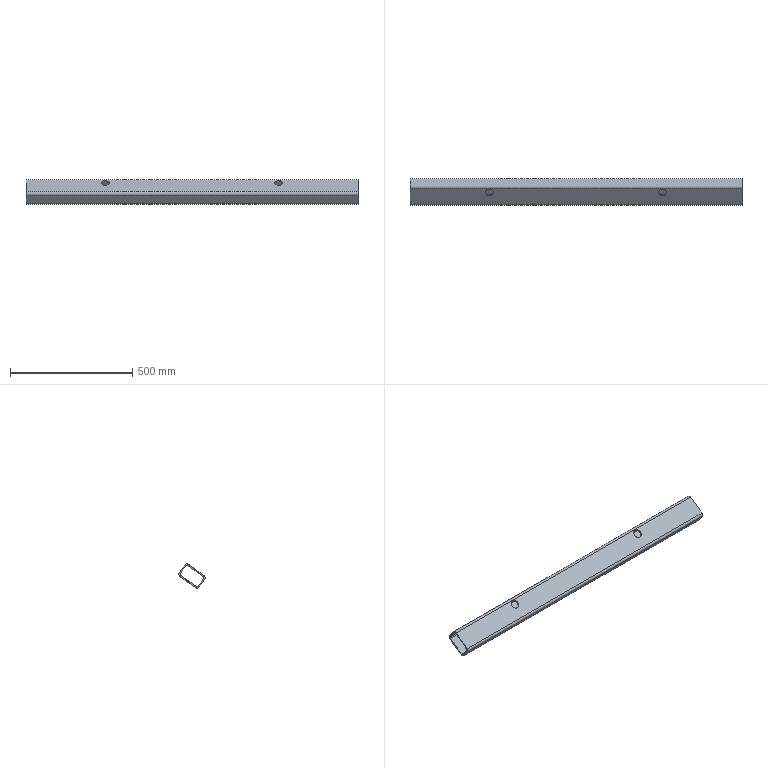Component | SolidWorks | Poprecna spona 1360mm-48 | 1 solid | 26 faces | box 1360 x 108.18 x 99.53 mm | volume 1934284 mm3 | cylinder 16 | plane 10 | commonest cylinder face diameters 34 x8 20 x4 10 x4 | material Plain Carbon Steel
build123d program:
from build123d import *

# Parameters (mm, degrees)
BOSS_EXTRUDE1_DEPTH      = 680
BOSS_EXTRUDE1_DEPTH_BACK = 680
SKETCH2_R                = 17
CUT_EXTRUDE1_DEPTH       = 685.471


with BuildPart() as part:
    # Sketch1 → Boss-Extrude1 (new, two sides: drawn at the far end of the back side and taken through both)
    with BuildSketch(Plane(origin=(0, 0, 0), x_dir=(0, 0, -1), z_dir=(1, 0, 0)).offset(-BOSS_EXTRUDE1_DEPTH_BACK)):
        with BuildLine():
            Line((-20, 50), (20, 50))
            ThreePointArc((20, 50), (27.071, 47.071), (30, 40))
            Line((30, 40), (30, -40))
            ThreePointArc((30, -40), (27.071, -47.071), (20, -50))
            Line((20, -50), (-20, -50))
            ThreePointArc((-20, -50), (-27.071, -47.071), (-30, -40))
            Line((-30, -40), (-30, 40))
            ThreePointArc((-30, 40), (-27.071, 47.071), (-20, 50))
        make_face()
        with BuildLine():
            Line((-25, 40), (-25, -40))
            ThreePointArc((-25, -40), (-23.536, -43.536), (-20, -45))
            Line((-20, -45), (20, -45))
            ThreePointArc((20, -45), (23.536, -43.536), (25, -40))
            Line((25, -40), (25, 40))
            ThreePointArc((25, 40), (23.536, 43.536), (20, 45))
            Line((20, 45), (-20, 45))
            ThreePointArc((-20, 45), (-23.536, 43.536), (-25, 40))
        make_face(mode=Mode.SUBTRACT)
    extrude(amount=BOSS_EXTRUDE1_DEPTH + BOSS_EXTRUDE1_DEPTH_BACK)

    # Sketch2 → Cut-Extrude1 (cut, through all)
    with BuildSketch(Plane.XY.offset(30)):
        with Locations((-355, 20)):
            Circle(SKETCH2_R)
    cut_extrude1 = extrude(amount=-CUT_EXTRUDE1_DEPTH, mode=Mode.SUBTRACT)

    # Mirror1: Cut-Extrude1 across plane
    add(cut_extrude1.mirror(Plane(origin=(0, 0, 0), x_dir=(0, 0, 1), z_dir=(1, 0, 0))), mode=Mode.SUBTRACT)


solid = part.part

# Placed as in the assembly
solid = solid.moved(Location((-633.6, 700.788, 236.028), (36.21, 0, 0)))
STEP:
#1=COLOUR_RGB('',0.7922,0.8196,0.9333);
#2=FILL_AREA_STYLE_COLOUR('',#1);
#3=FILL_AREA_STYLE('',(#2));
#4=SURFACE_STYLE_FILL_AREA(#3);
#5=SURFACE_SIDE_STYLE('',(#4));
#6=SURFACE_STYLE_USAGE(.BOTH.,#5);
#7=PRESENTATION_STYLE_ASSIGNMENT((#6));
#8=CARTESIAN_POINT('',(-10.299,28.923,8.805));
#9=VERTEX_POINT('',#8);
#10=CARTESIAN_POINT('',(-11.638,28.923,8.805));
#11=VERTEX_POINT('',#10);
#12=CARTESIAN_POINT('',(-10.969,28.923,8.805));
#13=DIRECTION('',(-0.,0.5907,-0.8069));
#14=DIRECTION('',(-1.,0.,0.));
#15=AXIS2_PLACEMENT_3D('',#12,#13,#14);
#16=CIRCLE('',#15,0.6693);
#17=EDGE_CURVE('',#9,#11,#16,.T.);
#18=ORIENTED_EDGE('',*,*,#17,.T.);
#19=CARTESIAN_POINT('',(-11.638,28.807,8.963));
#20=VERTEX_POINT('',#19);
#21=CARTESIAN_POINT('',(-11.638,28.923,8.805));
#22=DIRECTION('',(0.,-0.5907,0.8069));
#23=VECTOR('',#22,39.37);
#24=LINE('',#21,#23);
#25=EDGE_CURVE('',#11,#20,#24,.T.);
#26=ORIENTED_EDGE('',*,*,#25,.T.);
#27=CARTESIAN_POINT('',(-10.299,28.807,8.963));
#28=VERTEX_POINT('',#27);
#29=CARTESIAN_POINT('',(-10.969,28.807,8.963));
#30=DIRECTION('',(0.,-0.5907,0.8069));
#31=DIRECTION('',(0.,0.8069,0.5907));
#32=AXIS2_PLACEMENT_3D('',#29,#30,#31);
#33=CIRCLE('',#32,0.6693);
#34=EDGE_CURVE('',#20,#28,#33,.T.);
#35=ORIENTED_EDGE('',*,*,#34,.T.);
#36=CARTESIAN_POINT('',(-10.299,28.923,8.805));
#37=DIRECTION('',(0.,-0.5907,0.8069));
#38=VECTOR('',#37,39.37);
#39=LINE('',#36,#38);
#40=EDGE_CURVE('',#9,#28,#39,.T.);
#41=ORIENTED_EDGE('',*,*,#40,.F.);
#42=EDGE_LOOP('',(#18,#26,#35,#41));
#43=FACE_OUTER_BOUND('',#42,.T.);
#44=CARTESIAN_POINT('',(-10.969,28.923,8.805));
#45=DIRECTION('',(0.,-0.5907,0.8069));
#46=DIRECTION('',(1.,0.,0.));
#47=AXIS2_PLACEMENT_3D('',#44,#45,#46);
#48=CYLINDRICAL_SURFACE('',#47,0.6693);
#49=ADVANCED_FACE('',(#43),#48,.F.);
#50=CARTESIAN_POINT('',(-10.299,27.644,10.552));
#51=VERTEX_POINT('',#50);
#52=CARTESIAN_POINT('',(-11.638,27.644,10.552));
#53=VERTEX_POINT('',#52);
#54=CARTESIAN_POINT('',(-10.969,27.644,10.552));
#55=DIRECTION('',(-0.,0.5907,-0.8069));
#56=DIRECTION('',(1.,0.,0.));
#57=AXIS2_PLACEMENT_3D('',#54,#55,#56);
#58=CIRCLE('',#57,0.6693);
#59=EDGE_CURVE('',#51,#53,#58,.T.);
#60=ORIENTED_EDGE('',*,*,#59,.T.);
#61=CARTESIAN_POINT('',(-11.638,27.528,10.711));
#62=VERTEX_POINT('',#61);
#63=CARTESIAN_POINT('',(-11.638,28.923,8.805));
#64=DIRECTION('',(0.,-0.5907,0.8069));
#65=VECTOR('',#64,39.37);
#66=LINE('',#63,#65);
#67=EDGE_CURVE('',#53,#62,#66,.T.);
#68=ORIENTED_EDGE('',*,*,#67,.T.);
#69=CARTESIAN_POINT('',(-10.299,27.528,10.711));
#70=VERTEX_POINT('',#69);
#71=CARTESIAN_POINT('',(-10.969,27.528,10.711));
#72=DIRECTION('',(-0.,0.5907,-0.8069));
#73=DIRECTION('',(-1.,0.,0.));
#74=AXIS2_PLACEMENT_3D('',#71,#72,#73);
#75=CIRCLE('',#74,0.6693);
#76=EDGE_CURVE('',#70,#62,#75,.T.);
#77=ORIENTED_EDGE('',*,*,#76,.F.);
#78=CARTESIAN_POINT('',(-10.299,28.923,8.805));
#79=DIRECTION('',(0.,-0.5907,0.8069));
#80=VECTOR('',#79,39.37);
#81=LINE('',#78,#80);
#82=EDGE_CURVE('',#51,#70,#81,.T.);
#83=ORIENTED_EDGE('',*,*,#82,.F.);
#84=EDGE_LOOP('',(#60,#68,#77,#83));
#85=FACE_OUTER_BOUND('',#84,.T.);
#86=CARTESIAN_POINT('',(-10.969,28.923,8.805));
#87=DIRECTION('',(0.,-0.5907,0.8069));
#88=DIRECTION('',(1.,0.,0.));
#89=AXIS2_PLACEMENT_3D('',#86,#87,#88);
#90=CYLINDRICAL_SURFACE('',#89,0.6693);
#91=ADVANCED_FACE('',(#85),#90,.F.);
#92=CARTESIAN_POINT('',(-39.591,28.923,8.805));
#93=VERTEX_POINT('',#92);
#94=CARTESIAN_POINT('',(-38.252,28.923,8.805));
#95=VERTEX_POINT('',#94);
#96=CARTESIAN_POINT('',(-38.921,28.923,8.805));
#97=DIRECTION('',(0.,-0.5907,0.8069));
#98=DIRECTION('',(1.,0.,0.));
#99=AXIS2_PLACEMENT_3D('',#96,#97,#98);
#100=CIRCLE('',#99,0.6693);
#101=EDGE_CURVE('',#93,#95,#100,.T.);
#102=ORIENTED_EDGE('',*,*,#101,.F.);
#103=CARTESIAN_POINT('',(-39.591,28.807,8.963));
#104=VERTEX_POINT('',#103);
#105=CARTESIAN_POINT('',(-39.591,28.923,8.805));
#106=DIRECTION('',(0.,-0.5907,0.8069));
#107=VECTOR('',#106,39.37);
#108=LINE('',#105,#107);
#109=EDGE_CURVE('',#93,#104,#108,.T.);
#110=ORIENTED_EDGE('',*,*,#109,.T.);
#111=CARTESIAN_POINT('',(-38.252,28.807,8.963));
#112=VERTEX_POINT('',#111);
#113=CARTESIAN_POINT('',(-38.921,28.807,8.963));
#114=DIRECTION('',(-0.,0.5907,-0.8069));
#115=DIRECTION('',(0.,0.8069,0.5907));
#116=AXIS2_PLACEMENT_3D('',#113,#114,#115);
#117=CIRCLE('',#116,0.6693);
#118=EDGE_CURVE('',#112,#104,#117,.T.);
#119=ORIENTED_EDGE('',*,*,#118,.F.);
#120=CARTESIAN_POINT('',(-38.252,28.923,8.805));
#121=DIRECTION('',(0.,-0.5907,0.8069));
#122=VECTOR('',#121,39.37);
#123=LINE('',#120,#122);
#124=EDGE_CURVE('',#95,#112,#123,.T.);
#125=ORIENTED_EDGE('',*,*,#124,.F.);
#126=EDGE_LOOP('',(#102,#110,#119,#125));
#127=FACE_OUTER_BOUND('',#126,.T.);
#128=CARTESIAN_POINT('',(-38.921,28.923,8.805));
#129=DIRECTION('',(0.,-0.5907,0.8069));
#130=DIRECTION('',(1.,0.,0.));
#131=AXIS2_PLACEMENT_3D('',#128,#129,#130);
#132=CYLINDRICAL_SURFACE('',#131,0.6693);
#133=ADVANCED_FACE('',(#127),#132,.F.);
#134=CARTESIAN_POINT('',(-39.591,27.644,10.552));
#135=VERTEX_POINT('',#134);
#136=CARTESIAN_POINT('',(-38.252,27.644,10.552));
#137=VERTEX_POINT('',#136);
#138=CARTESIAN_POINT('',(-38.921,27.644,10.552));
#139=DIRECTION('',(0.,-0.5907,0.8069));
#140=DIRECTION('',(1.,0.,0.));
#141=AXIS2_PLACEMENT_3D('',#138,#139,#140);
#142=CIRCLE('',#141,0.6693);
#143=EDGE_CURVE('',#135,#137,#142,.T.);
#144=ORIENTED_EDGE('',*,*,#143,.F.);
#145=CARTESIAN_POINT('',(-39.591,27.528,10.711));
#146=VERTEX_POINT('',#145);
#147=CARTESIAN_POINT('',(-39.591,28.923,8.805));
#148=DIRECTION('',(0.,-0.5907,0.8069));
#149=VECTOR('',#148,39.37);
#150=LINE('',#147,#149);
#151=EDGE_CURVE('',#135,#146,#150,.T.);
#152=ORIENTED_EDGE('',*,*,#151,.T.);
#153=CARTESIAN_POINT('',(-38.252,27.528,10.711));
#154=VERTEX_POINT('',#153);
#155=CARTESIAN_POINT('',(-38.921,27.528,10.711));
#156=DIRECTION('',(0.,-0.5907,0.8069));
#157=DIRECTION('',(1.,0.,0.));
#158=AXIS2_PLACEMENT_3D('',#155,#156,#157);
#159=CIRCLE('',#158,0.6693);
#160=EDGE_CURVE('',#146,#154,#159,.T.);
#161=ORIENTED_EDGE('',*,*,#160,.T.);
#162=CARTESIAN_POINT('',(-38.252,28.923,8.805));
#163=DIRECTION('',(0.,-0.5907,0.8069));
#164=VECTOR('',#163,39.37);
#165=LINE('',#162,#164);
#166=EDGE_CURVE('',#137,#154,#165,.T.);
#167=ORIENTED_EDGE('',*,*,#166,.F.);
#168=EDGE_LOOP('',(#144,#152,#161,#167));
#169=FACE_OUTER_BOUND('',#168,.T.);
#170=CARTESIAN_POINT('',(-38.921,28.923,8.805));
#171=DIRECTION('',(0.,-0.5907,0.8069));
#172=DIRECTION('',(1.,0.,0.));
#173=AXIS2_PLACEMENT_3D('',#170,#171,#172);
#174=CYLINDRICAL_SURFACE('',#173,0.6693);
#175=ADVANCED_FACE('',(#169),#174,.F.);
#176=CARTESIAN_POINT('',(-51.717,25.537,8.765));
#177=VERTEX_POINT('',#176);
#178=CARTESIAN_POINT('',(1.827,25.537,8.765));
#179=VERTEX_POINT('',#178);
#180=CARTESIAN_POINT('',(-51.717,25.537,8.765));
#181=DIRECTION('',(1.,-0.,-0.));
#182=VECTOR('',#181,39.37);
#183=LINE('',#180,#182);
#184=EDGE_CURVE('',#177,#179,#183,.T.);
#185=ORIENTED_EDGE('',*,*,#184,.T.);
#186=CARTESIAN_POINT('',(1.827,25.622,9.315));
#187=VERTEX_POINT('',#186);
#188=CARTESIAN_POINT('',(1.827,25.854,8.997));
#189=DIRECTION('',(1.,-0.,-0.));
#190=DIRECTION('',(0.,0.5907,-0.8069));
#191=AXIS2_PLACEMENT_3D('',#188,#189,#190);
#192=CIRCLE('',#191,0.3937);
#193=EDGE_CURVE('',#187,#179,#192,.T.);
#194=ORIENTED_EDGE('',*,*,#193,.F.);
#195=CARTESIAN_POINT('',(-51.717,25.622,9.315));
#196=VERTEX_POINT('',#195);
#197=CARTESIAN_POINT('',(-51.717,25.622,9.315));
#198=DIRECTION('',(1.,-0.,-0.));
#199=VECTOR('',#198,39.37);
#200=LINE('',#197,#199);
#201=EDGE_CURVE('',#196,#187,#200,.T.);
#202=ORIENTED_EDGE('',*,*,#201,.F.);
#203=CARTESIAN_POINT('',(-51.717,25.854,8.997));
#204=DIRECTION('',(1.,-0.,-0.));
#205=DIRECTION('',(0.,0.5907,-0.8069));
#206=AXIS2_PLACEMENT_3D('',#203,#204,#205);
#207=CIRCLE('',#206,0.3937);
#208=EDGE_CURVE('',#196,#177,#207,.T.);
#209=ORIENTED_EDGE('',*,*,#208,.T.);
#210=EDGE_LOOP('',(#185,#194,#202,#209));
#211=FACE_OUTER_BOUND('',#210,.T.);
#212=CARTESIAN_POINT('',(-51.717,25.854,8.997));
#213=DIRECTION('',(1.,-0.,-0.));
#214=DIRECTION('',(0.,0.5907,-0.8069));
#215=AXIS2_PLACEMENT_3D('',#212,#213,#214);
#216=CYLINDRICAL_SURFACE('',#215,0.3937);
#217=ADVANCED_FACE('',(#211),#216,.T.);
#218=ORIENTED_EDGE('',*,*,#76,.T.);
#219=CARTESIAN_POINT('',(-10.969,27.528,10.711));
#220=DIRECTION('',(-0.,0.5907,-0.8069));
#221=DIRECTION('',(-1.,0.,0.));
#222=AXIS2_PLACEMENT_3D('',#219,#220,#221);
#223=CIRCLE('',#222,0.6693);
#224=EDGE_CURVE('',#62,#70,#223,.T.);
#225=ORIENTED_EDGE('',*,*,#224,.T.);
#226=EDGE_LOOP('',(#218,#225));
#227=FACE_BOUND('',#226,.T.);
#228=CARTESIAN_POINT('',(-38.921,27.528,10.711));
#229=DIRECTION('',(0.,-0.5907,0.8069));
#230=DIRECTION('',(1.,0.,0.));
#231=AXIS2_PLACEMENT_3D('',#228,#229,#230);
#232=CIRCLE('',#231,0.6693);
#233=EDGE_CURVE('',#154,#146,#232,.T.);
#234=ORIENTED_EDGE('',*,*,#233,.F.);
#235=ORIENTED_EDGE('',*,*,#160,.F.);
#236=EDGE_LOOP('',(#234,#235));
#237=FACE_BOUND('',#236,.T.);
#238=ORIENTED_EDGE('',*,*,#201,.T.);
#239=CARTESIAN_POINT('',(1.827,28.163,11.176));
#240=VERTEX_POINT('',#239);
#241=CARTESIAN_POINT('',(1.827,28.163,11.176));
#242=DIRECTION('',(-0.,-0.8069,-0.5907));
#243=VECTOR('',#242,39.37);
#244=LINE('',#241,#243);
#245=EDGE_CURVE('',#240,#187,#244,.T.);
#246=ORIENTED_EDGE('',*,*,#245,.F.);
#247=CARTESIAN_POINT('',(-51.717,28.163,11.176));
#248=VERTEX_POINT('',#247);
#249=CARTESIAN_POINT('',(-51.717,28.163,11.176));
#250=DIRECTION('',(1.,-0.,-0.));
#251=VECTOR('',#250,39.37);
#252=LINE('',#249,#251);
#253=EDGE_CURVE('',#248,#240,#252,.T.);
#254=ORIENTED_EDGE('',*,*,#253,.F.);
#255=CARTESIAN_POINT('',(-51.717,28.163,11.176));
#256=DIRECTION('',(-0.,-0.8069,-0.5907));
#257=VECTOR('',#256,39.37);
#258=LINE('',#255,#257);
#259=EDGE_CURVE('',#248,#196,#258,.T.);
#260=ORIENTED_EDGE('',*,*,#259,.T.);
#261=EDGE_LOOP('',(#238,#246,#254,#260));
#262=FACE_OUTER_BOUND('',#261,.T.);
#263=CARTESIAN_POINT('',(-51.717,28.163,11.176));
#264=DIRECTION('',(0.,-0.5907,0.8069));
#265=DIRECTION('',(-0.,-0.8069,-0.5907));
#266=AXIS2_PLACEMENT_3D('',#263,#264,#265);
#267=PLANE('',#266);
#268=ADVANCED_FACE('',(#227,#237,#262),#267,.T.);
#269=ORIENTED_EDGE('',*,*,#253,.T.);
#270=CARTESIAN_POINT('',(1.827,28.713,11.091));
#271=VERTEX_POINT('',#270);
#272=CARTESIAN_POINT('',(1.827,28.396,10.858));
#273=DIRECTION('',(1.,-0.,-0.));
#274=DIRECTION('',(0.,0.5907,-0.8069));
#275=AXIS2_PLACEMENT_3D('',#272,#273,#274);
#276=CIRCLE('',#275,0.3937);
#277=EDGE_CURVE('',#271,#240,#276,.T.);
#278=ORIENTED_EDGE('',*,*,#277,.F.);
#279=CARTESIAN_POINT('',(-51.717,28.713,11.091));
#280=VERTEX_POINT('',#279);
#281=CARTESIAN_POINT('',(-51.717,28.713,11.091));
#282=DIRECTION('',(1.,-0.,-0.));
#283=VECTOR('',#282,39.37);
#284=LINE('',#281,#283);
#285=EDGE_CURVE('',#280,#271,#284,.T.);
#286=ORIENTED_EDGE('',*,*,#285,.F.);
#287=CARTESIAN_POINT('',(-51.717,28.396,10.858));
#288=DIRECTION('',(1.,-0.,-0.));
#289=DIRECTION('',(0.,0.5907,-0.8069));
#290=AXIS2_PLACEMENT_3D('',#287,#288,#289);
#291=CIRCLE('',#290,0.3937);
#292=EDGE_CURVE('',#280,#248,#291,.T.);
#293=ORIENTED_EDGE('',*,*,#292,.T.);
#294=EDGE_LOOP('',(#269,#278,#286,#293));
#295=FACE_OUTER_BOUND('',#294,.T.);
#296=CARTESIAN_POINT('',(-51.717,28.396,10.858));
#297=DIRECTION('',(1.,-0.,-0.));
#298=DIRECTION('',(0.,0.5907,-0.8069));
#299=AXIS2_PLACEMENT_3D('',#296,#297,#298);
#300=CYLINDRICAL_SURFACE('',#299,0.3937);
#301=ADVANCED_FACE('',(#295),#300,.T.);
#302=ORIENTED_EDGE('',*,*,#285,.T.);
#303=CARTESIAN_POINT('',(1.827,29.644,9.82));
#304=VERTEX_POINT('',#303);
#305=CARTESIAN_POINT('',(1.827,28.713,11.091));
#306=DIRECTION('',(0.,-0.5907,0.8069));
#307=VECTOR('',#306,39.37);
#308=LINE('',#305,#307);
#309=EDGE_CURVE('',#304,#271,#308,.T.);
#310=ORIENTED_EDGE('',*,*,#309,.F.);
#311=CARTESIAN_POINT('',(-51.717,29.644,9.82));
#312=VERTEX_POINT('',#311);
#313=CARTESIAN_POINT('',(-51.717,29.644,9.82));
#314=DIRECTION('',(1.,-0.,-0.));
#315=VECTOR('',#314,39.37);
#316=LINE('',#313,#315);
#317=EDGE_CURVE('',#312,#304,#316,.T.);
#318=ORIENTED_EDGE('',*,*,#317,.F.);
#319=CARTESIAN_POINT('',(-51.717,28.713,11.091));
#320=DIRECTION('',(0.,-0.5907,0.8069));
#321=VECTOR('',#320,39.37);
#322=LINE('',#319,#321);
#323=EDGE_CURVE('',#312,#280,#322,.T.);
#324=ORIENTED_EDGE('',*,*,#323,.T.);
#325=EDGE_LOOP('',(#302,#310,#318,#324));
#326=FACE_OUTER_BOUND('',#325,.T.);
#327=CARTESIAN_POINT('',(-51.717,28.713,11.091));
#328=DIRECTION('',(0.,0.8069,0.5907));
#329=DIRECTION('',(0.,-0.5907,0.8069));
#330=AXIS2_PLACEMENT_3D('',#327,#328,#329);
#331=PLANE('',#330);
#332=ADVANCED_FACE('',(#326),#331,.T.);
#333=ORIENTED_EDGE('',*,*,#317,.T.);
#334=CARTESIAN_POINT('',(1.827,29.558,9.27));
#335=VERTEX_POINT('',#334);
#336=CARTESIAN_POINT('',(1.827,29.326,9.587));
#337=DIRECTION('',(1.,-0.,-0.));
#338=DIRECTION('',(0.,-0.5907,0.8069));
#339=AXIS2_PLACEMENT_3D('',#336,#337,#338);
#340=CIRCLE('',#339,0.3937);
#341=EDGE_CURVE('',#335,#304,#340,.T.);
#342=ORIENTED_EDGE('',*,*,#341,.F.);
#343=CARTESIAN_POINT('',(-51.717,29.558,9.27));
#344=VERTEX_POINT('',#343);
#345=CARTESIAN_POINT('',(-51.717,29.558,9.27));
#346=DIRECTION('',(1.,-0.,-0.));
#347=VECTOR('',#346,39.37);
#348=LINE('',#345,#347);
#349=EDGE_CURVE('',#344,#335,#348,.T.);
#350=ORIENTED_EDGE('',*,*,#349,.F.);
#351=CARTESIAN_POINT('',(-51.717,29.326,9.587));
#352=DIRECTION('',(1.,-0.,-0.));
#353=DIRECTION('',(0.,-0.5907,0.8069));
#354=AXIS2_PLACEMENT_3D('',#351,#352,#353);
#355=CIRCLE('',#354,0.3937);
#356=EDGE_CURVE('',#344,#312,#355,.T.);
#357=ORIENTED_EDGE('',*,*,#356,.T.);
#358=EDGE_LOOP('',(#333,#342,#350,#357));
#359=FACE_OUTER_BOUND('',#358,.T.);
#360=CARTESIAN_POINT('',(-51.717,29.326,9.587));
#361=DIRECTION('',(1.,-0.,-0.));
#362=DIRECTION('',(0.,0.5907,-0.8069));
#363=AXIS2_PLACEMENT_3D('',#360,#361,#362);
#364=CYLINDRICAL_SURFACE('',#363,0.3937);
#365=ADVANCED_FACE('',(#359),#364,.T.);
#366=ORIENTED_EDGE('',*,*,#17,.F.);
#367=CARTESIAN_POINT('',(-10.969,28.923,8.805));
#368=DIRECTION('',(-0.,0.5907,-0.8069));
#369=DIRECTION('',(-1.,0.,0.));
#370=AXIS2_PLACEMENT_3D('',#367,#368,#369);
#371=CIRCLE('',#370,0.6693);
#372=EDGE_CURVE('',#11,#9,#371,.T.);
#373=ORIENTED_EDGE('',*,*,#372,.F.);
#374=EDGE_LOOP('',(#366,#373));
#375=FACE_BOUND('',#374,.T.);
#376=CARTESIAN_POINT('',(-38.921,28.923,8.805));
#377=DIRECTION('',(0.,-0.5907,0.8069));
#378=DIRECTION('',(1.,0.,0.));
#379=AXIS2_PLACEMENT_3D('',#376,#377,#378);
#380=CIRCLE('',#379,0.6693);
#381=EDGE_CURVE('',#95,#93,#380,.T.);
#382=ORIENTED_EDGE('',*,*,#381,.T.);
#383=ORIENTED_EDGE('',*,*,#101,.T.);
#384=EDGE_LOOP('',(#382,#383));
#385=FACE_BOUND('',#384,.T.);
#386=ORIENTED_EDGE('',*,*,#349,.T.);
#387=CARTESIAN_POINT('',(1.827,27.017,7.409));
#388=VERTEX_POINT('',#387);
#389=CARTESIAN_POINT('',(1.827,29.558,9.27));
#390=DIRECTION('',(0.,0.8069,0.5907));
#391=VECTOR('',#390,39.37);
#392=LINE('',#389,#391);
#393=EDGE_CURVE('',#388,#335,#392,.T.);
#394=ORIENTED_EDGE('',*,*,#393,.F.);
#395=CARTESIAN_POINT('',(-51.717,27.017,7.409));
#396=VERTEX_POINT('',#395);
#397=CARTESIAN_POINT('',(-51.717,27.017,7.409));
#398=DIRECTION('',(1.,-0.,-0.));
#399=VECTOR('',#398,39.37);
#400=LINE('',#397,#399);
#401=EDGE_CURVE('',#396,#388,#400,.T.);
#402=ORIENTED_EDGE('',*,*,#401,.F.);
#403=CARTESIAN_POINT('',(-51.717,29.558,9.27));
#404=DIRECTION('',(0.,0.8069,0.5907));
#405=VECTOR('',#404,39.37);
#406=LINE('',#403,#405);
#407=EDGE_CURVE('',#396,#344,#406,.T.);
#408=ORIENTED_EDGE('',*,*,#407,.T.);
#409=EDGE_LOOP('',(#386,#394,#402,#408));
#410=FACE_OUTER_BOUND('',#409,.T.);
#411=CARTESIAN_POINT('',(-51.717,29.558,9.27));
#412=DIRECTION('',(-0.,0.5907,-0.8069));
#413=DIRECTION('',(0.,0.8069,0.5907));
#414=AXIS2_PLACEMENT_3D('',#411,#412,#413);
#415=PLANE('',#414);
#416=ADVANCED_FACE('',(#375,#385,#410),#415,.T.);
#417=ORIENTED_EDGE('',*,*,#401,.T.);
#418=CARTESIAN_POINT('',(1.827,26.467,7.494));
#419=VERTEX_POINT('',#418);
#420=CARTESIAN_POINT('',(1.827,26.785,7.727));
#421=DIRECTION('',(1.,-0.,-0.));
#422=DIRECTION('',(0.,0.5907,-0.8069));
#423=AXIS2_PLACEMENT_3D('',#420,#421,#422);
#424=CIRCLE('',#423,0.3937);
#425=EDGE_CURVE('',#419,#388,#424,.T.);
#426=ORIENTED_EDGE('',*,*,#425,.F.);
#427=CARTESIAN_POINT('',(-51.717,26.467,7.494));
#428=VERTEX_POINT('',#427);
#429=CARTESIAN_POINT('',(-51.717,26.467,7.494));
#430=DIRECTION('',(1.,-0.,-0.));
#431=VECTOR('',#430,39.37);
#432=LINE('',#429,#431);
#433=EDGE_CURVE('',#428,#419,#432,.T.);
#434=ORIENTED_EDGE('',*,*,#433,.F.);
#435=CARTESIAN_POINT('',(-51.717,26.785,7.727));
#436=DIRECTION('',(1.,-0.,-0.));
#437=DIRECTION('',(0.,0.5907,-0.8069));
#438=AXIS2_PLACEMENT_3D('',#435,#436,#437);
#439=CIRCLE('',#438,0.3937);
#440=EDGE_CURVE('',#428,#396,#439,.T.);
#441=ORIENTED_EDGE('',*,*,#440,.T.);
#442=EDGE_LOOP('',(#417,#426,#434,#441));
#443=FACE_OUTER_BOUND('',#442,.T.);
#444=CARTESIAN_POINT('',(-51.717,26.785,7.727));
#445=DIRECTION('',(1.,-0.,-0.));
#446=DIRECTION('',(0.,0.5907,-0.8069));
#447=AXIS2_PLACEMENT_3D('',#444,#445,#446);
#448=CYLINDRICAL_SURFACE('',#447,0.3937);
#449=ADVANCED_FACE('',(#443),#448,.T.);
#450=ORIENTED_EDGE('',*,*,#433,.T.);
#451=CARTESIAN_POINT('',(1.827,25.537,8.765));
#452=DIRECTION('',(-0.,0.5907,-0.8069));
#453=VECTOR('',#452,39.37);
#454=LINE('',#451,#453);
#455=EDGE_CURVE('',#179,#419,#454,.T.);
#456=ORIENTED_EDGE('',*,*,#455,.F.);
#457=ORIENTED_EDGE('',*,*,#184,.F.);
#458=CARTESIAN_POINT('',(-51.717,25.537,8.765));
#459=DIRECTION('',(-0.,0.5907,-0.8069));
#460=VECTOR('',#459,39.37);
#461=LINE('',#458,#460);
#462=EDGE_CURVE('',#177,#428,#461,.T.);
#463=ORIENTED_EDGE('',*,*,#462,.T.);
#464=EDGE_LOOP('',(#450,#456,#457,#463));
#465=FACE_OUTER_BOUND('',#464,.T.);
#466=CARTESIAN_POINT('',(-51.717,25.537,8.765));
#467=DIRECTION('',(-0.,-0.8069,-0.5907));
#468=DIRECTION('',(-0.,0.5907,-0.8069));
#469=AXIS2_PLACEMENT_3D('',#466,#467,#468);
#470=PLANE('',#469);
#471=ADVANCED_FACE('',(#465),#470,.T.);
#472=CARTESIAN_POINT('',(-51.717,29.485,9.704));
#473=VERTEX_POINT('',#472);
#474=CARTESIAN_POINT('',(-51.717,28.554,10.974));
#475=VERTEX_POINT('',#474);
#476=CARTESIAN_POINT('',(-51.717,28.554,10.974));
#477=DIRECTION('',(0.,-0.5907,0.8069));
#478=VECTOR('',#477,39.37);
#479=LINE('',#476,#478);
#480=EDGE_CURVE('',#473,#475,#479,.T.);
#481=ORIENTED_EDGE('',*,*,#480,.T.);
#482=CARTESIAN_POINT('',(-51.717,28.279,11.017));
#483=VERTEX_POINT('',#482);
#484=CARTESIAN_POINT('',(-51.717,28.396,10.858));
#485=DIRECTION('',(1.,-0.,-0.));
#486=DIRECTION('',(0.,0.5907,-0.8069));
#487=AXIS2_PLACEMENT_3D('',#484,#485,#486);
#488=CIRCLE('',#487,0.1969);
#489=EDGE_CURVE('',#475,#483,#488,.T.);
#490=ORIENTED_EDGE('',*,*,#489,.T.);
#491=CARTESIAN_POINT('',(-51.717,25.738,9.156));
#492=VERTEX_POINT('',#491);
#493=CARTESIAN_POINT('',(-51.717,28.279,11.017));
#494=DIRECTION('',(-0.,-0.8069,-0.5907));
#495=VECTOR('',#494,39.37);
#496=LINE('',#493,#495);
#497=EDGE_CURVE('',#483,#492,#496,.T.);
#498=ORIENTED_EDGE('',*,*,#497,.T.);
#499=CARTESIAN_POINT('',(-51.717,25.695,8.881));
#500=VERTEX_POINT('',#499);
#501=CARTESIAN_POINT('',(-51.717,25.854,8.997));
#502=DIRECTION('',(1.,-0.,-0.));
#503=DIRECTION('',(0.,0.5907,-0.8069));
#504=AXIS2_PLACEMENT_3D('',#501,#502,#503);
#505=CIRCLE('',#504,0.1969);
#506=EDGE_CURVE('',#492,#500,#505,.T.);
#507=ORIENTED_EDGE('',*,*,#506,.T.);
#508=CARTESIAN_POINT('',(-51.717,26.626,7.611));
#509=VERTEX_POINT('',#508);
#510=CARTESIAN_POINT('',(-51.717,25.695,8.881));
#511=DIRECTION('',(-0.,0.5907,-0.8069));
#512=VECTOR('',#511,39.37);
#513=LINE('',#510,#512);
#514=EDGE_CURVE('',#500,#509,#513,.T.);
#515=ORIENTED_EDGE('',*,*,#514,.T.);
#516=CARTESIAN_POINT('',(-51.717,26.901,7.568));
#517=VERTEX_POINT('',#516);
#518=CARTESIAN_POINT('',(-51.717,26.785,7.727));
#519=DIRECTION('',(1.,-0.,-0.));
#520=DIRECTION('',(0.,0.5907,-0.8069));
#521=AXIS2_PLACEMENT_3D('',#518,#519,#520);
#522=CIRCLE('',#521,0.1969);
#523=EDGE_CURVE('',#509,#517,#522,.T.);
#524=ORIENTED_EDGE('',*,*,#523,.T.);
#525=CARTESIAN_POINT('',(-51.717,29.442,9.429));
#526=VERTEX_POINT('',#525);
#527=CARTESIAN_POINT('',(-51.717,29.442,9.429));
#528=DIRECTION('',(0.,0.8069,0.5907));
#529=VECTOR('',#528,39.37);
#530=LINE('',#527,#529);
#531=EDGE_CURVE('',#517,#526,#530,.T.);
#532=ORIENTED_EDGE('',*,*,#531,.T.);
#533=CARTESIAN_POINT('',(-51.717,29.326,9.587));
#534=DIRECTION('',(1.,-0.,-0.));
#535=DIRECTION('',(0.,-0.5907,0.8069));
#536=AXIS2_PLACEMENT_3D('',#533,#534,#535);
#537=CIRCLE('',#536,0.1969);
#538=EDGE_CURVE('',#526,#473,#537,.T.);
#539=ORIENTED_EDGE('',*,*,#538,.T.);
#540=EDGE_LOOP('',(#481,#490,#498,#507,#515,#524,#532,#539));
#541=FACE_BOUND('',#540,.T.);
#542=ORIENTED_EDGE('',*,*,#208,.F.);
#543=ORIENTED_EDGE('',*,*,#259,.F.);
#544=ORIENTED_EDGE('',*,*,#292,.F.);
#545=ORIENTED_EDGE('',*,*,#323,.F.);
#546=ORIENTED_EDGE('',*,*,#356,.F.);
#547=ORIENTED_EDGE('',*,*,#407,.F.);
#548=ORIENTED_EDGE('',*,*,#440,.F.);
#549=ORIENTED_EDGE('',*,*,#462,.F.);
#550=EDGE_LOOP('',(#542,#543,#544,#545,#546,#547,#548,#549));
#551=FACE_OUTER_BOUND('',#550,.T.);
#552=CARTESIAN_POINT('',(-51.717,25.854,8.997));
#553=DIRECTION('',(1.,-0.,-0.));
#554=DIRECTION('',(-0.,0.5907,-0.8069));
#555=AXIS2_PLACEMENT_3D('',#552,#553,#554);
#556=PLANE('',#555);
#557=ADVANCED_FACE('',(#541,#551),#556,.F.);
#558=CARTESIAN_POINT('',(1.827,28.554,10.974));
#559=VERTEX_POINT('',#558);
#560=CARTESIAN_POINT('',(-51.717,28.554,10.974));
#561=DIRECTION('',(1.,-0.,-0.));
#562=VECTOR('',#561,39.37);
#563=LINE('',#560,#562);
#564=EDGE_CURVE('',#475,#559,#563,.T.);
#565=ORIENTED_EDGE('',*,*,#564,.T.);
#566=CARTESIAN_POINT('',(1.827,28.279,11.017));
#567=VERTEX_POINT('',#566);
#568=CARTESIAN_POINT('',(1.827,28.396,10.858));
#569=DIRECTION('',(1.,-0.,-0.));
#570=DIRECTION('',(0.,0.5907,-0.8069));
#571=AXIS2_PLACEMENT_3D('',#568,#569,#570);
#572=CIRCLE('',#571,0.1969);
#573=EDGE_CURVE('',#559,#567,#572,.T.);
#574=ORIENTED_EDGE('',*,*,#573,.T.);
#575=CARTESIAN_POINT('',(-51.717,28.279,11.017));
#576=DIRECTION('',(1.,-0.,-0.));
#577=VECTOR('',#576,39.37);
#578=LINE('',#575,#577);
#579=EDGE_CURVE('',#483,#567,#578,.T.);
#580=ORIENTED_EDGE('',*,*,#579,.F.);
#581=ORIENTED_EDGE('',*,*,#489,.F.);
#582=EDGE_LOOP('',(#565,#574,#580,#581));
#583=FACE_OUTER_BOUND('',#582,.T.);
#584=CARTESIAN_POINT('',(-51.717,28.396,10.858));
#585=DIRECTION('',(1.,-0.,-0.));
#586=DIRECTION('',(0.,0.5907,-0.8069));
#587=AXIS2_PLACEMENT_3D('',#584,#585,#586);
#588=CYLINDRICAL_SURFACE('',#587,0.1969);
#589=ADVANCED_FACE('',(#583),#588,.F.);
#590=CARTESIAN_POINT('',(1.827,29.485,9.704));
#591=VERTEX_POINT('',#590);
#592=CARTESIAN_POINT('',(-51.717,29.485,9.704));
#593=DIRECTION('',(1.,-0.,-0.));
#594=VECTOR('',#593,39.37);
#595=LINE('',#592,#594);
#596=EDGE_CURVE('',#473,#591,#595,.T.);
#597=ORIENTED_EDGE('',*,*,#596,.T.);
#598=CARTESIAN_POINT('',(1.827,28.554,10.974));
#599=DIRECTION('',(0.,-0.5907,0.8069));
#600=VECTOR('',#599,39.37);
#601=LINE('',#598,#600);
#602=EDGE_CURVE('',#591,#559,#601,.T.);
#603=ORIENTED_EDGE('',*,*,#602,.T.);
#604=ORIENTED_EDGE('',*,*,#564,.F.);
#605=ORIENTED_EDGE('',*,*,#480,.F.);
#606=EDGE_LOOP('',(#597,#603,#604,#605));
#607=FACE_OUTER_BOUND('',#606,.T.);
#608=CARTESIAN_POINT('',(-51.717,28.554,10.974));
#609=DIRECTION('',(0.,0.8069,0.5907));
#610=DIRECTION('',(0.,-0.5907,0.8069));
#611=AXIS2_PLACEMENT_3D('',#608,#609,#610);
#612=PLANE('',#611);
#613=ADVANCED_FACE('',(#607),#612,.F.);
#614=CARTESIAN_POINT('',(1.827,29.442,9.429));
#615=VERTEX_POINT('',#614);
#616=CARTESIAN_POINT('',(-51.717,29.442,9.429));
#617=DIRECTION('',(1.,-0.,-0.));
#618=VECTOR('',#617,39.37);
#619=LINE('',#616,#618);
#620=EDGE_CURVE('',#526,#615,#619,.T.);
#621=ORIENTED_EDGE('',*,*,#620,.T.);
#622=CARTESIAN_POINT('',(1.827,29.326,9.587));
#623=DIRECTION('',(1.,-0.,-0.));
#624=DIRECTION('',(0.,-0.5907,0.8069));
#625=AXIS2_PLACEMENT_3D('',#622,#623,#624);
#626=CIRCLE('',#625,0.1969);
#627=EDGE_CURVE('',#615,#591,#626,.T.);
#628=ORIENTED_EDGE('',*,*,#627,.T.);
#629=ORIENTED_EDGE('',*,*,#596,.F.);
#630=ORIENTED_EDGE('',*,*,#538,.F.);
#631=EDGE_LOOP('',(#621,#628,#629,#630));
#632=FACE_OUTER_BOUND('',#631,.T.);
#633=CARTESIAN_POINT('',(-51.717,29.326,9.587));
#634=DIRECTION('',(1.,-0.,-0.));
#635=DIRECTION('',(0.,0.5907,-0.8069));
#636=AXIS2_PLACEMENT_3D('',#633,#634,#635);
#637=CYLINDRICAL_SURFACE('',#636,0.1969);
#638=ADVANCED_FACE('',(#632),#637,.F.);
#639=CARTESIAN_POINT('',(-10.969,28.807,8.963));
#640=DIRECTION('',(0.,-0.5907,0.8069));
#641=DIRECTION('',(-0.,0.8069,0.5907));
#642=AXIS2_PLACEMENT_3D('',#639,#640,#641);
#643=CIRCLE('',#642,0.6693);
#644=EDGE_CURVE('',#28,#20,#643,.T.);
#645=ORIENTED_EDGE('',*,*,#644,.F.);
#646=ORIENTED_EDGE('',*,*,#34,.F.);
#647=EDGE_LOOP('',(#645,#646));
#648=FACE_BOUND('',#647,.T.);
#649=ORIENTED_EDGE('',*,*,#118,.T.);
#650=CARTESIAN_POINT('',(-38.921,28.807,8.963));
#651=DIRECTION('',(-0.,0.5907,-0.8069));
#652=DIRECTION('',(0.,0.8069,0.5907));
#653=AXIS2_PLACEMENT_3D('',#650,#651,#652);
#654=CIRCLE('',#653,0.6693);
#655=EDGE_CURVE('',#104,#112,#654,.T.);
#656=ORIENTED_EDGE('',*,*,#655,.T.);
#657=EDGE_LOOP('',(#649,#656));
#658=FACE_BOUND('',#657,.T.);
#659=CARTESIAN_POINT('',(1.827,26.901,7.568));
#660=VERTEX_POINT('',#659);
#661=CARTESIAN_POINT('',(-51.717,26.901,7.568));
#662=DIRECTION('',(1.,-0.,-0.));
#663=VECTOR('',#662,39.37);
#664=LINE('',#661,#663);
#665=EDGE_CURVE('',#517,#660,#664,.T.);
#666=ORIENTED_EDGE('',*,*,#665,.T.);
#667=CARTESIAN_POINT('',(1.827,29.442,9.429));
#668=DIRECTION('',(0.,0.8069,0.5907));
#669=VECTOR('',#668,39.37);
#670=LINE('',#667,#669);
#671=EDGE_CURVE('',#660,#615,#670,.T.);
#672=ORIENTED_EDGE('',*,*,#671,.T.);
#673=ORIENTED_EDGE('',*,*,#620,.F.);
#674=ORIENTED_EDGE('',*,*,#531,.F.);
#675=EDGE_LOOP('',(#666,#672,#673,#674));
#676=FACE_OUTER_BOUND('',#675,.T.);
#677=CARTESIAN_POINT('',(-51.717,29.442,9.429));
#678=DIRECTION('',(-0.,0.5907,-0.8069));
#679=DIRECTION('',(0.,0.8069,0.5907));
#680=AXIS2_PLACEMENT_3D('',#677,#678,#679);
#681=PLANE('',#680);
#682=ADVANCED_FACE('',(#648,#658,#676),#681,.F.);
#683=CARTESIAN_POINT('',(1.827,26.626,7.611));
#684=VERTEX_POINT('',#683);
#685=CARTESIAN_POINT('',(-51.717,26.626,7.611));
#686=DIRECTION('',(1.,-0.,-0.));
#687=VECTOR('',#686,39.37);
#688=LINE('',#685,#687);
#689=EDGE_CURVE('',#509,#684,#688,.T.);
#690=ORIENTED_EDGE('',*,*,#689,.T.);
#691=CARTESIAN_POINT('',(1.827,26.785,7.727));
#692=DIRECTION('',(1.,-0.,-0.));
#693=DIRECTION('',(0.,0.5907,-0.8069));
#694=AXIS2_PLACEMENT_3D('',#691,#692,#693);
#695=CIRCLE('',#694,0.1969);
#696=EDGE_CURVE('',#684,#660,#695,.T.);
#697=ORIENTED_EDGE('',*,*,#696,.T.);
#698=ORIENTED_EDGE('',*,*,#665,.F.);
#699=ORIENTED_EDGE('',*,*,#523,.F.);
#700=EDGE_LOOP('',(#690,#697,#698,#699));
#701=FACE_OUTER_BOUND('',#700,.T.);
#702=CARTESIAN_POINT('',(-51.717,26.785,7.727));
#703=DIRECTION('',(1.,-0.,-0.));
#704=DIRECTION('',(0.,0.5907,-0.8069));
#705=AXIS2_PLACEMENT_3D('',#702,#703,#704);
#706=CYLINDRICAL_SURFACE('',#705,0.1969);
#707=ADVANCED_FACE('',(#701),#706,.F.);
#708=CARTESIAN_POINT('',(1.827,25.695,8.881));
#709=VERTEX_POINT('',#708);
#710=CARTESIAN_POINT('',(-51.717,25.695,8.881));
#711=DIRECTION('',(1.,-0.,-0.));
#712=VECTOR('',#711,39.37);
#713=LINE('',#710,#712);
#714=EDGE_CURVE('',#500,#709,#713,.T.);
#715=ORIENTED_EDGE('',*,*,#714,.T.);
#716=CARTESIAN_POINT('',(1.827,25.695,8.881));
#717=DIRECTION('',(-0.,0.5907,-0.8069));
#718=VECTOR('',#717,39.37);
#719=LINE('',#716,#718);
#720=EDGE_CURVE('',#709,#684,#719,.T.);
#721=ORIENTED_EDGE('',*,*,#720,.T.);
#722=ORIENTED_EDGE('',*,*,#689,.F.);
#723=ORIENTED_EDGE('',*,*,#514,.F.);
#724=EDGE_LOOP('',(#715,#721,#722,#723));
#725=FACE_OUTER_BOUND('',#724,.T.);
#726=CARTESIAN_POINT('',(-51.717,25.695,8.881));
#727=DIRECTION('',(-0.,-0.8069,-0.5907));
#728=DIRECTION('',(-0.,0.5907,-0.8069));
#729=AXIS2_PLACEMENT_3D('',#726,#727,#728);
#730=PLANE('',#729);
#731=ADVANCED_FACE('',(#725),#730,.F.);
#732=CARTESIAN_POINT('',(1.827,25.738,9.156));
#733=VERTEX_POINT('',#732);
#734=CARTESIAN_POINT('',(-51.717,25.738,9.156));
#735=DIRECTION('',(1.,-0.,-0.));
#736=VECTOR('',#735,39.37);
#737=LINE('',#734,#736);
#738=EDGE_CURVE('',#492,#733,#737,.T.);
#739=ORIENTED_EDGE('',*,*,#738,.T.);
#740=CARTESIAN_POINT('',(1.827,25.854,8.997));
#741=DIRECTION('',(1.,-0.,-0.));
#742=DIRECTION('',(0.,0.5907,-0.8069));
#743=AXIS2_PLACEMENT_3D('',#740,#741,#742);
#744=CIRCLE('',#743,0.1969);
#745=EDGE_CURVE('',#733,#709,#744,.T.);
#746=ORIENTED_EDGE('',*,*,#745,.T.);
#747=ORIENTED_EDGE('',*,*,#714,.F.);
#748=ORIENTED_EDGE('',*,*,#506,.F.);
#749=EDGE_LOOP('',(#739,#746,#747,#748));
#750=FACE_OUTER_BOUND('',#749,.T.);
#751=CARTESIAN_POINT('',(-51.717,25.854,8.997));
#752=DIRECTION('',(1.,-0.,-0.));
#753=DIRECTION('',(0.,0.5907,-0.8069));
#754=AXIS2_PLACEMENT_3D('',#751,#752,#753);
#755=CYLINDRICAL_SURFACE('',#754,0.1969);
#756=ADVANCED_FACE('',(#750),#755,.F.);
#757=ORIENTED_EDGE('',*,*,#59,.F.);
#758=CARTESIAN_POINT('',(-10.969,27.644,10.552));
#759=DIRECTION('',(-0.,0.5907,-0.8069));
#760=DIRECTION('',(1.,0.,0.));
#761=AXIS2_PLACEMENT_3D('',#758,#759,#760);
#762=CIRCLE('',#761,0.6693);
#763=EDGE_CURVE('',#53,#51,#762,.T.);
#764=ORIENTED_EDGE('',*,*,#763,.F.);
#765=EDGE_LOOP('',(#757,#764));
#766=FACE_BOUND('',#765,.T.);
#767=CARTESIAN_POINT('',(-38.921,27.644,10.552));
#768=DIRECTION('',(0.,-0.5907,0.8069));
#769=DIRECTION('',(1.,0.,0.));
#770=AXIS2_PLACEMENT_3D('',#767,#768,#769);
#771=CIRCLE('',#770,0.6693);
#772=EDGE_CURVE('',#137,#135,#771,.T.);
#773=ORIENTED_EDGE('',*,*,#772,.T.);
#774=ORIENTED_EDGE('',*,*,#143,.T.);
#775=EDGE_LOOP('',(#773,#774));
#776=FACE_BOUND('',#775,.T.);
#777=ORIENTED_EDGE('',*,*,#579,.T.);
#778=CARTESIAN_POINT('',(1.827,28.279,11.017));
#779=DIRECTION('',(-0.,-0.8069,-0.5907));
#780=VECTOR('',#779,39.37);
#781=LINE('',#778,#780);
#782=EDGE_CURVE('',#567,#733,#781,.T.);
#783=ORIENTED_EDGE('',*,*,#782,.T.);
#784=ORIENTED_EDGE('',*,*,#738,.F.);
#785=ORIENTED_EDGE('',*,*,#497,.F.);
#786=EDGE_LOOP('',(#777,#783,#784,#785));
#787=FACE_OUTER_BOUND('',#786,.T.);
#788=CARTESIAN_POINT('',(-51.717,28.279,11.017));
#789=DIRECTION('',(0.,-0.5907,0.8069));
#790=DIRECTION('',(1.,-0.,-0.));
#791=AXIS2_PLACEMENT_3D('',#788,#789,#790);
#792=PLANE('',#791);
#793=ADVANCED_FACE('',(#766,#776,#787),#792,.F.);
#794=ORIENTED_EDGE('',*,*,#193,.T.);
#795=ORIENTED_EDGE('',*,*,#455,.T.);
#796=ORIENTED_EDGE('',*,*,#425,.T.);
#797=ORIENTED_EDGE('',*,*,#393,.T.);
#798=ORIENTED_EDGE('',*,*,#341,.T.);
#799=ORIENTED_EDGE('',*,*,#309,.T.);
#800=ORIENTED_EDGE('',*,*,#277,.T.);
#801=ORIENTED_EDGE('',*,*,#245,.T.);
#802=EDGE_LOOP('',(#794,#795,#796,#797,#798,#799,#800,#801));
#803=FACE_OUTER_BOUND('',#802,.T.);
#804=ORIENTED_EDGE('',*,*,#782,.F.);
#805=ORIENTED_EDGE('',*,*,#573,.F.);
#806=ORIENTED_EDGE('',*,*,#602,.F.);
#807=ORIENTED_EDGE('',*,*,#627,.F.);
#808=ORIENTED_EDGE('',*,*,#671,.F.);
#809=ORIENTED_EDGE('',*,*,#696,.F.);
#810=ORIENTED_EDGE('',*,*,#720,.F.);
#811=ORIENTED_EDGE('',*,*,#745,.F.);
#812=EDGE_LOOP('',(#804,#805,#806,#807,#808,#809,#810,#811));
#813=FACE_BOUND('',#812,.T.);
#814=CARTESIAN_POINT('',(1.827,25.854,8.997));
#815=DIRECTION('',(1.,-0.,-0.));
#816=DIRECTION('',(-0.,0.5907,-0.8069));
#817=AXIS2_PLACEMENT_3D('',#814,#815,#816);
#818=PLANE('',#817);
#819=ADVANCED_FACE('',(#803,#813),#818,.T.);
#820=ORIENTED_EDGE('',*,*,#151,.F.);
#821=ORIENTED_EDGE('',*,*,#772,.F.);
#822=ORIENTED_EDGE('',*,*,#166,.T.);
#823=ORIENTED_EDGE('',*,*,#233,.T.);
#824=EDGE_LOOP('',(#820,#821,#822,#823));
#825=FACE_OUTER_BOUND('',#824,.T.);
#826=CARTESIAN_POINT('',(-38.921,28.923,8.805));
#827=DIRECTION('',(0.,-0.5907,0.8069));
#828=DIRECTION('',(1.,0.,0.));
#829=AXIS2_PLACEMENT_3D('',#826,#827,#828);
#830=CYLINDRICAL_SURFACE('',#829,0.6693);
#831=ADVANCED_FACE('',(#825),#830,.F.);
#832=ORIENTED_EDGE('',*,*,#109,.F.);
#833=ORIENTED_EDGE('',*,*,#381,.F.);
#834=ORIENTED_EDGE('',*,*,#124,.T.);
#835=ORIENTED_EDGE('',*,*,#655,.F.);
#836=EDGE_LOOP('',(#832,#833,#834,#835));
#837=FACE_OUTER_BOUND('',#836,.T.);
#838=CARTESIAN_POINT('',(-38.921,28.923,8.805));
#839=DIRECTION('',(0.,-0.5907,0.8069));
#840=DIRECTION('',(1.,0.,0.));
#841=AXIS2_PLACEMENT_3D('',#838,#839,#840);
#842=CYLINDRICAL_SURFACE('',#841,0.6693);
#843=ADVANCED_FACE('',(#837),#842,.F.);
#844=ORIENTED_EDGE('',*,*,#67,.F.);
#845=ORIENTED_EDGE('',*,*,#763,.T.);
#846=ORIENTED_EDGE('',*,*,#82,.T.);
#847=ORIENTED_EDGE('',*,*,#224,.F.);
#848=EDGE_LOOP('',(#844,#845,#846,#847));
#849=FACE_OUTER_BOUND('',#848,.T.);
#850=CARTESIAN_POINT('',(-10.969,28.923,8.805));
#851=DIRECTION('',(0.,-0.5907,0.8069));
#852=DIRECTION('',(1.,0.,0.));
#853=AXIS2_PLACEMENT_3D('',#850,#851,#852);
#854=CYLINDRICAL_SURFACE('',#853,0.6693);
#855=ADVANCED_FACE('',(#849),#854,.F.);
#856=ORIENTED_EDGE('',*,*,#25,.F.);
#857=ORIENTED_EDGE('',*,*,#372,.T.);
#858=ORIENTED_EDGE('',*,*,#40,.T.);
#859=ORIENTED_EDGE('',*,*,#644,.T.);
#860=EDGE_LOOP('',(#856,#857,#858,#859));
#861=FACE_OUTER_BOUND('',#860,.T.);
#862=CARTESIAN_POINT('',(-10.969,28.923,8.805));
#863=DIRECTION('',(0.,-0.5907,0.8069));
#864=DIRECTION('',(1.,0.,0.));
#865=AXIS2_PLACEMENT_3D('',#862,#863,#864);
#866=CYLINDRICAL_SURFACE('',#865,0.6693);
#867=ADVANCED_FACE('',(#861),#866,.F.);
#868=CLOSED_SHELL('',(#49,#91,#133,#175,#217,#268,#301,#332,#365,#416,#449,#471,#557,#589,#613,#638,#682,#707,#731,#756,#793,#819,#831,#843,#855,#867));
#869=MANIFOLD_SOLID_BREP('',#868);
#870=STYLED_ITEM('',(#7),#869);
#871=(LENGTH_UNIT()NAMED_UNIT(*)SI_UNIT($,.METRE.));
#872=LENGTH_MEASURE_WITH_UNIT(LENGTH_MEASURE(0.0254),#871);
#873=DIMENSIONAL_EXPONENTS(1.,0.,0.,0.,0.,0.,0.);
#874=(CONVERSION_BASED_UNIT('',#872)LENGTH_UNIT()NAMED_UNIT(#873));
#875=UNCERTAINTY_MEASURE_WITH_UNIT(LENGTH_MEASURE(0.00001),#874,'','');
#876=(NAMED_UNIT(*)PLANE_ANGLE_UNIT()SI_UNIT($,.RADIAN.));
#877=(NAMED_UNIT(*)SI_UNIT($,.STERADIAN.)SOLID_ANGLE_UNIT());
#878=(GEOMETRIC_REPRESENTATION_CONTEXT(3)GLOBAL_UNCERTAINTY_ASSIGNED_CONTEXT((#875))GLOBAL_UNIT_ASSIGNED_CONTEXT((#874,#876,#877))REPRESENTATION_CONTEXT('',''));
#879=MECHANICAL_DESIGN_GEOMETRIC_PRESENTATION_REPRESENTATION('',(#870),#878);
#880=PRESENTATION_LAYER_ASSIGNMENT('','',(#870));
#881=CARTESIAN_POINT('',(0.,0.,0.));
#882=DIRECTION('',(0.,0.,1.));
#883=DIRECTION('',(1.,0.,0.));
#884=AXIS2_PLACEMENT_3D('',#881,#882,#883);
#885=(LENGTH_UNIT()NAMED_UNIT(*)SI_UNIT($,.METRE.));
#886=LENGTH_MEASURE_WITH_UNIT(LENGTH_MEASURE(0.0254),#885);
#887=DIMENSIONAL_EXPONENTS(1.,0.,0.,0.,0.,0.,0.);
#888=(CONVERSION_BASED_UNIT('',#886)LENGTH_UNIT()NAMED_UNIT(#887));
#889=UNCERTAINTY_MEASURE_WITH_UNIT(LENGTH_MEASURE(0.00001),#888,'','');
#890=(NAMED_UNIT(*)PLANE_ANGLE_UNIT()SI_UNIT($,.RADIAN.));
#891=(NAMED_UNIT(*)SI_UNIT($,.STERADIAN.)SOLID_ANGLE_UNIT());
#892=(GEOMETRIC_REPRESENTATION_CONTEXT(3)GLOBAL_UNCERTAINTY_ASSIGNED_CONTEXT((#889))GLOBAL_UNIT_ASSIGNED_CONTEXT((#888,#890,#891))REPRESENTATION_CONTEXT('',''));
#893=ADVANCED_BREP_SHAPE_REPRESENTATION('',(#869,#884),#892);